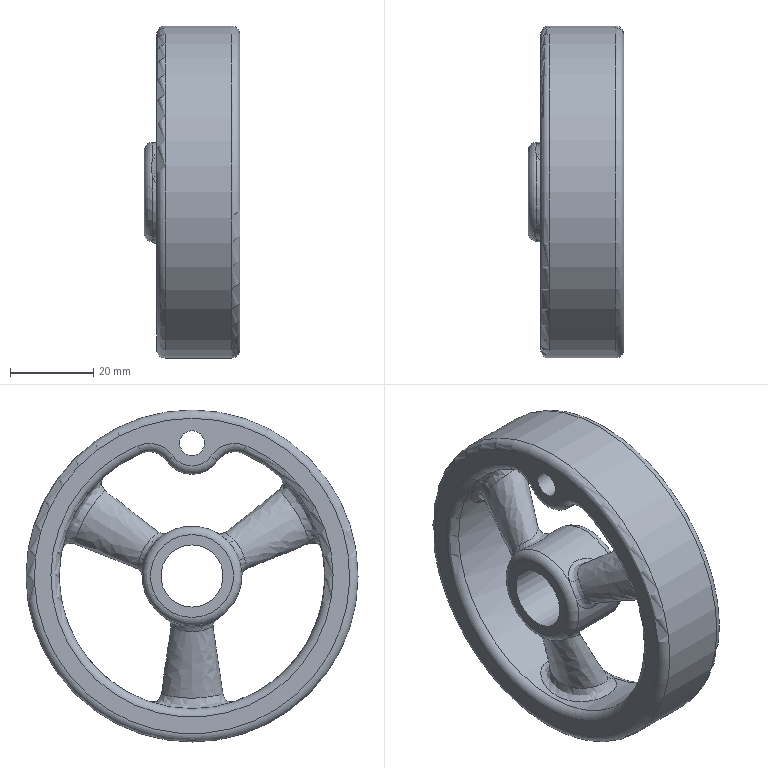Component | NX | HANDWHEEL_2 | 1 solid | 41 faces | volume 47494 mm3 | spline 15 | torus 12 | cylinder 9 | plane 5 | commonest cylinder face diameters 15 x2 10 x2 24 x1 80 x1 64 x1 19 x1 6 x1